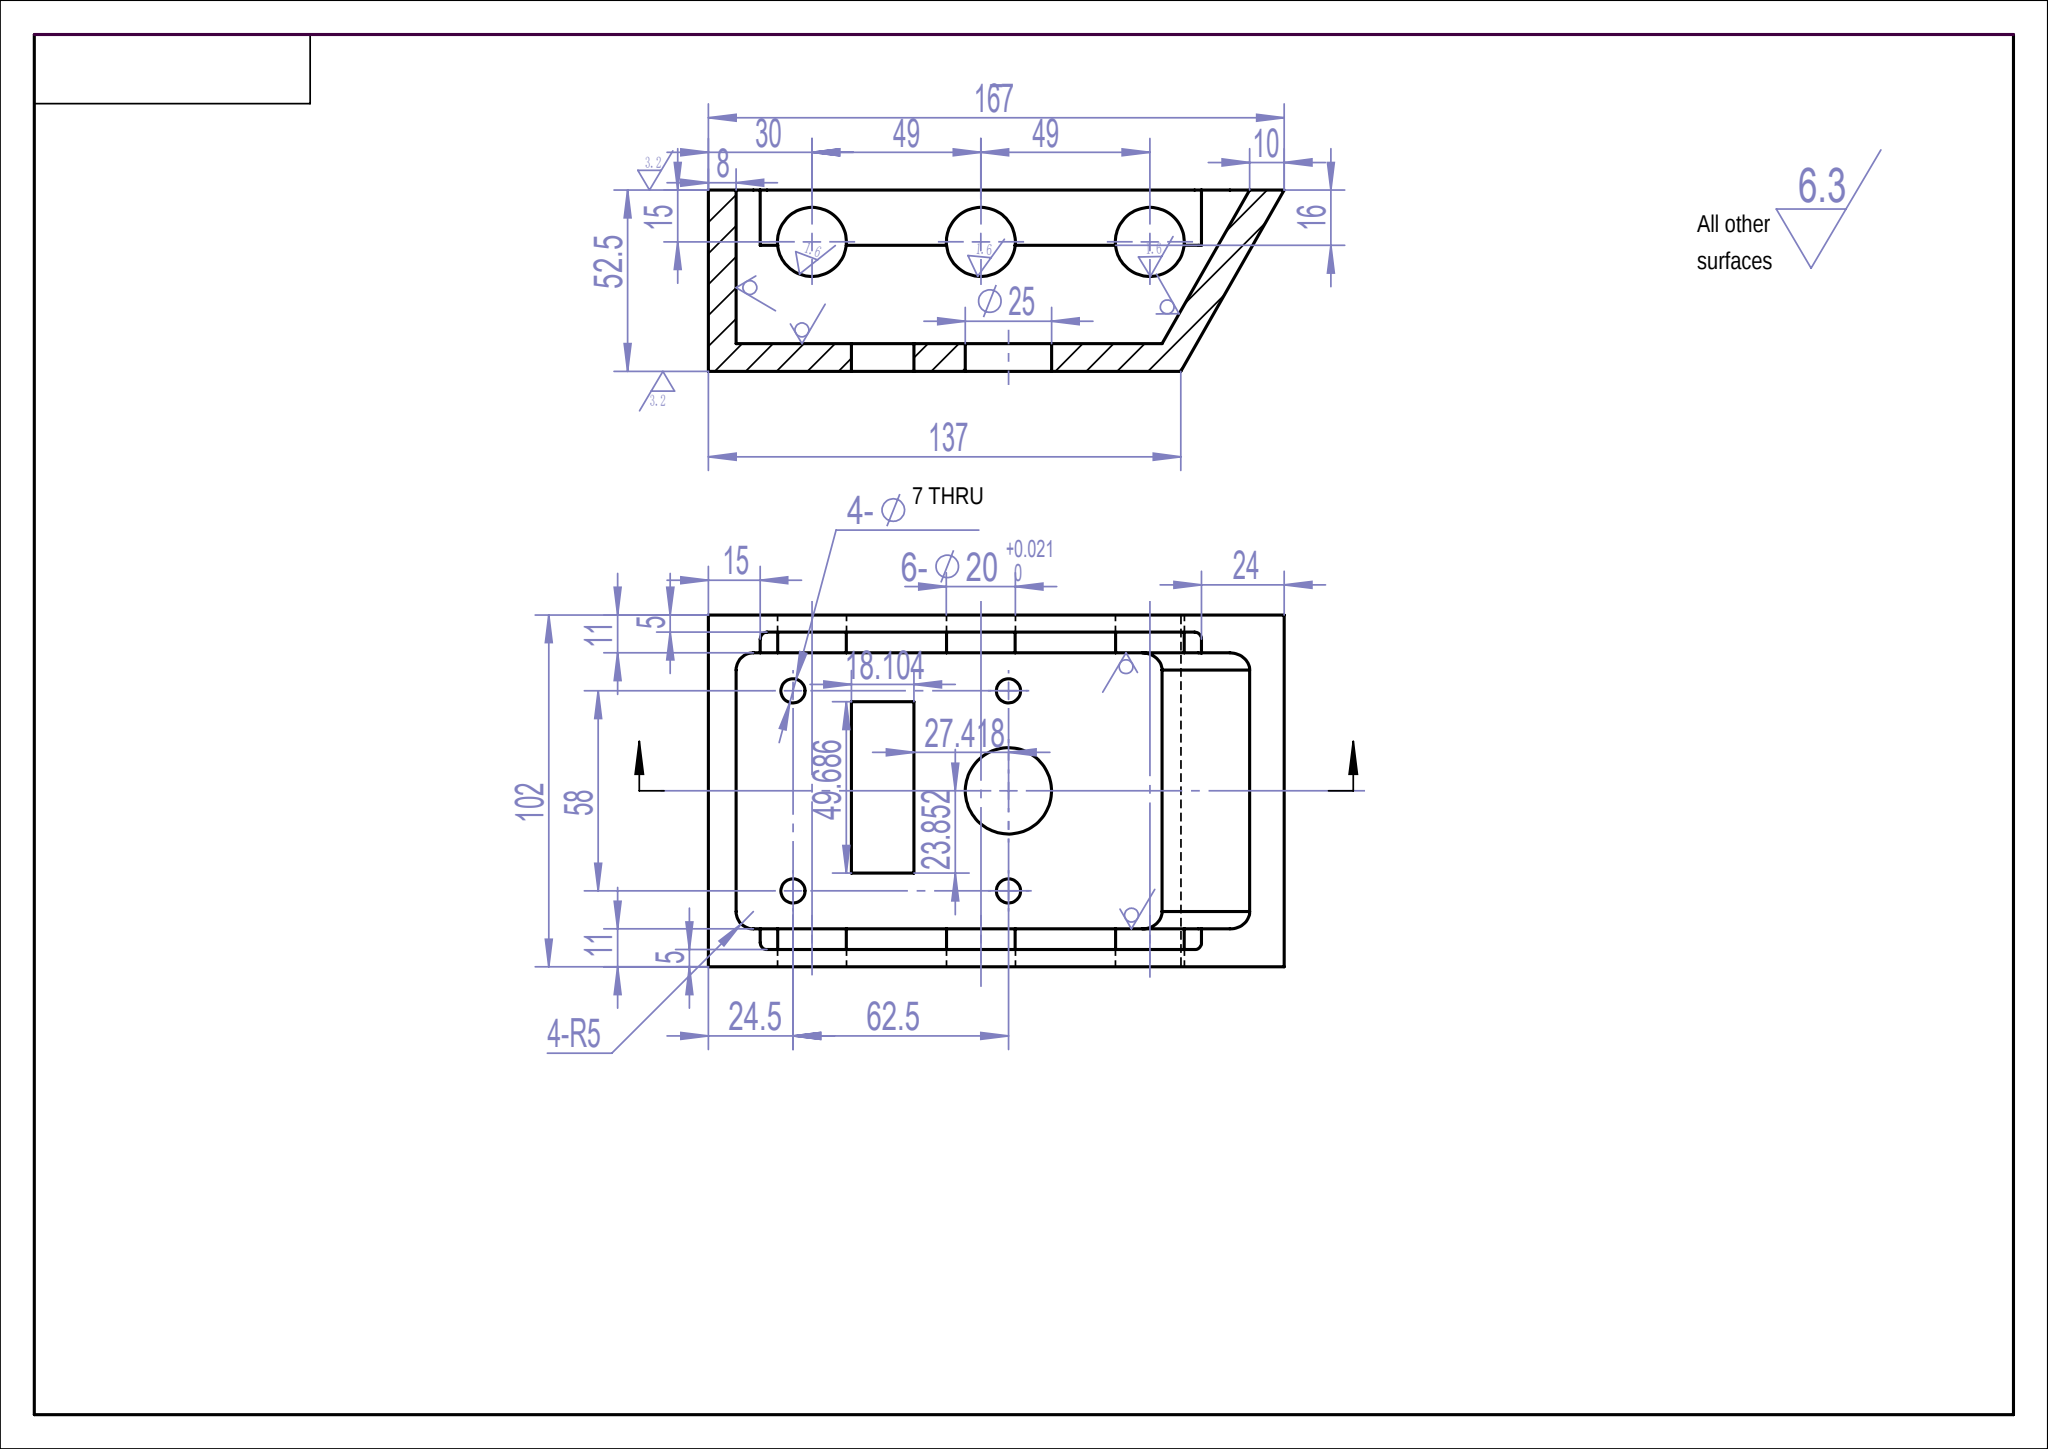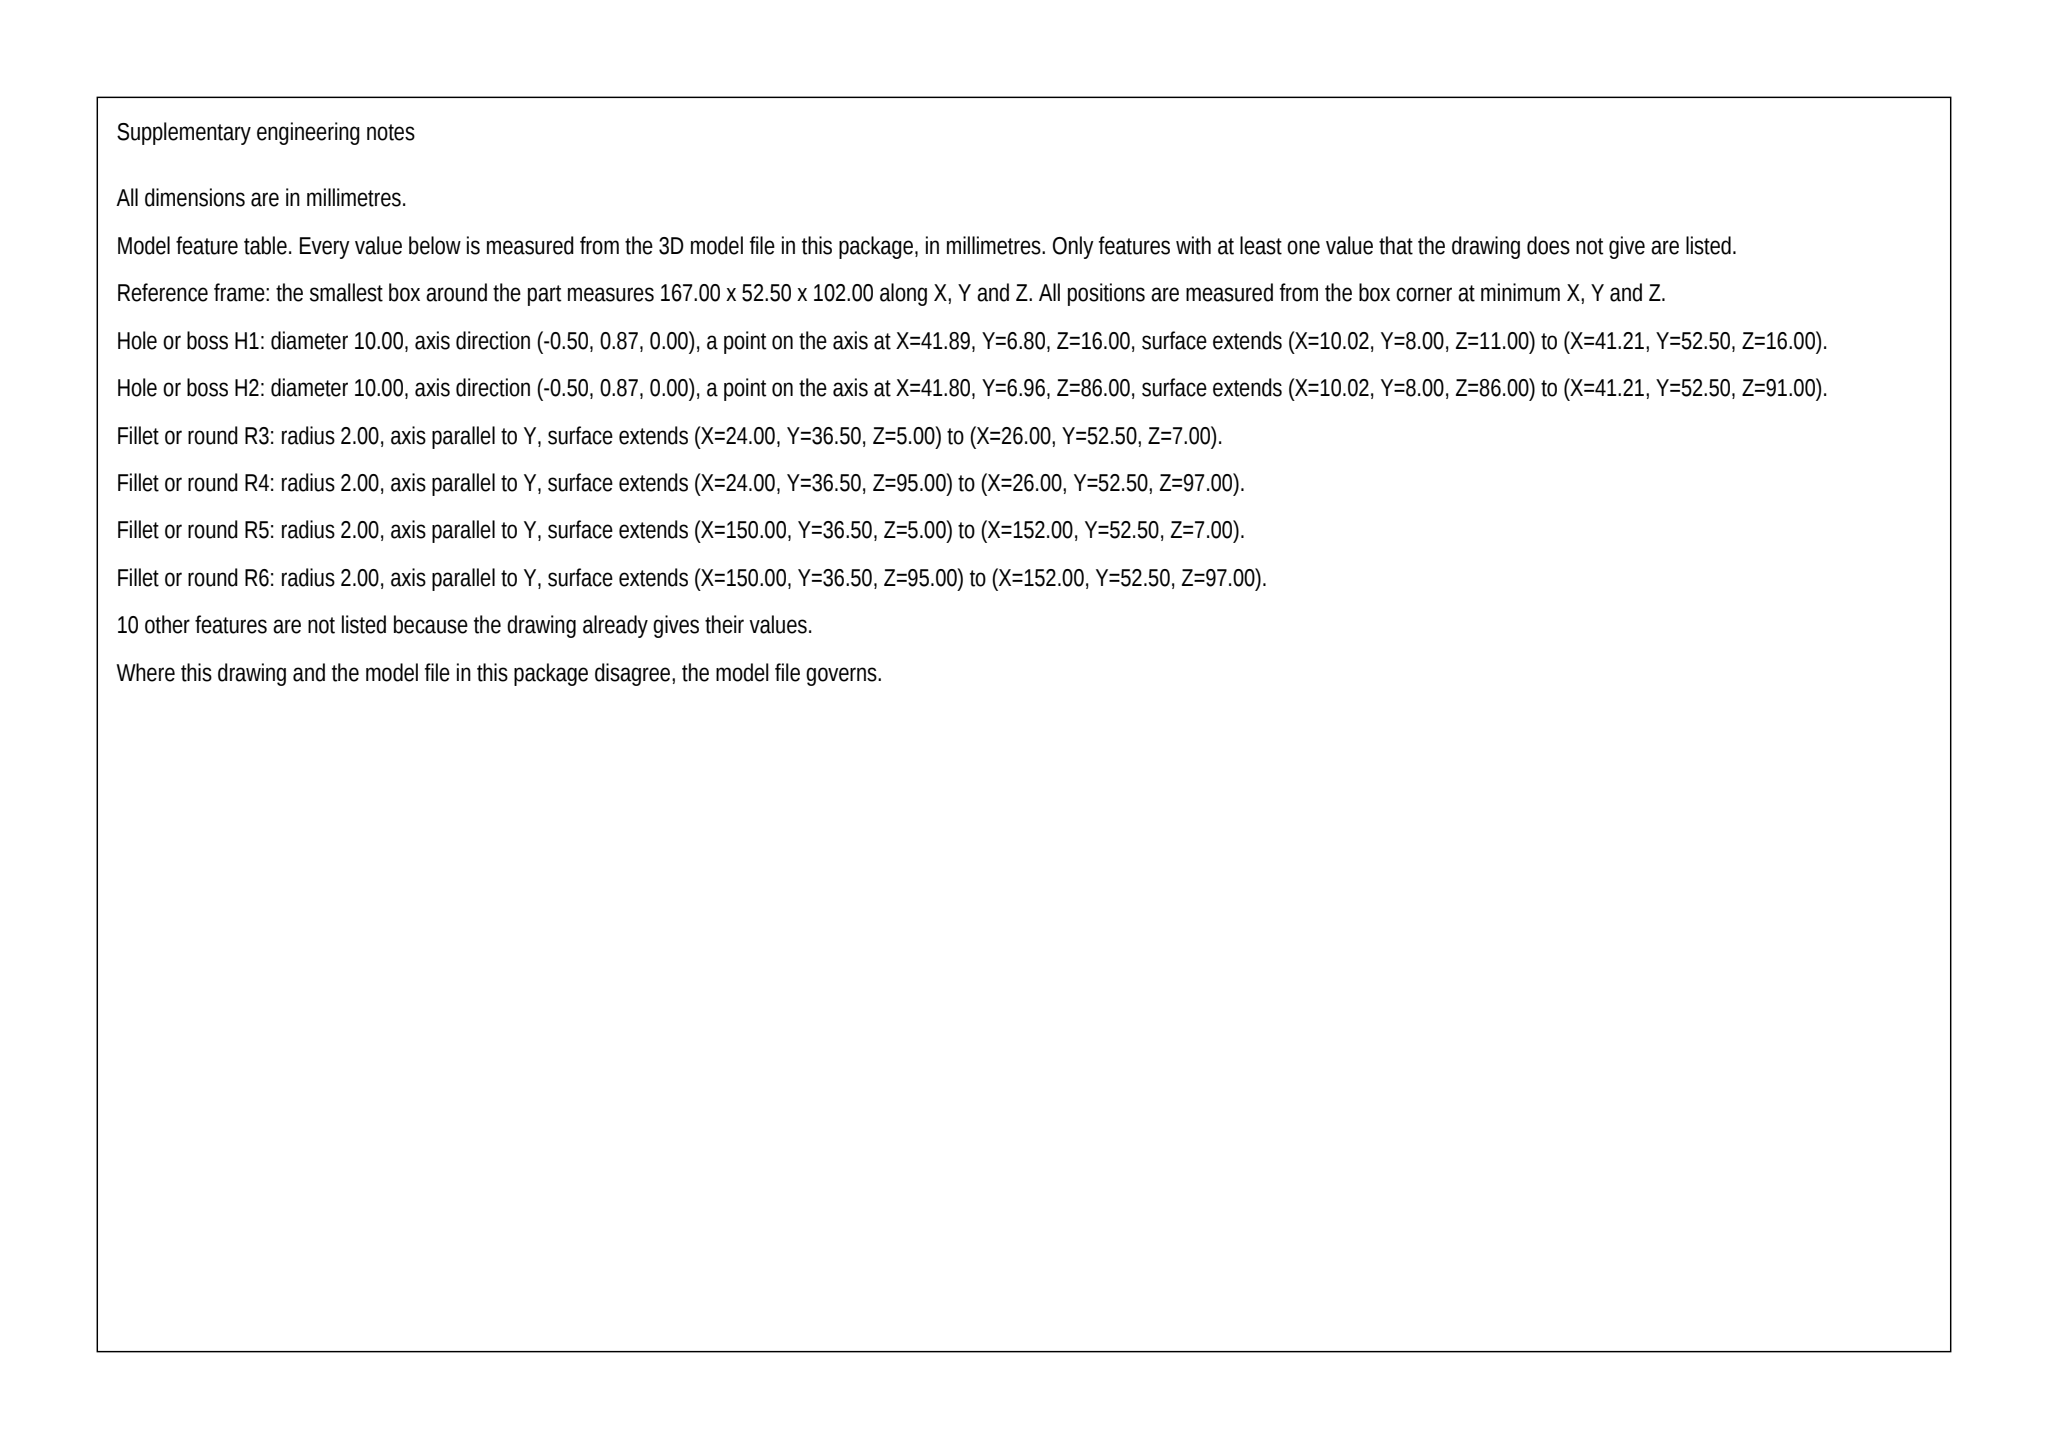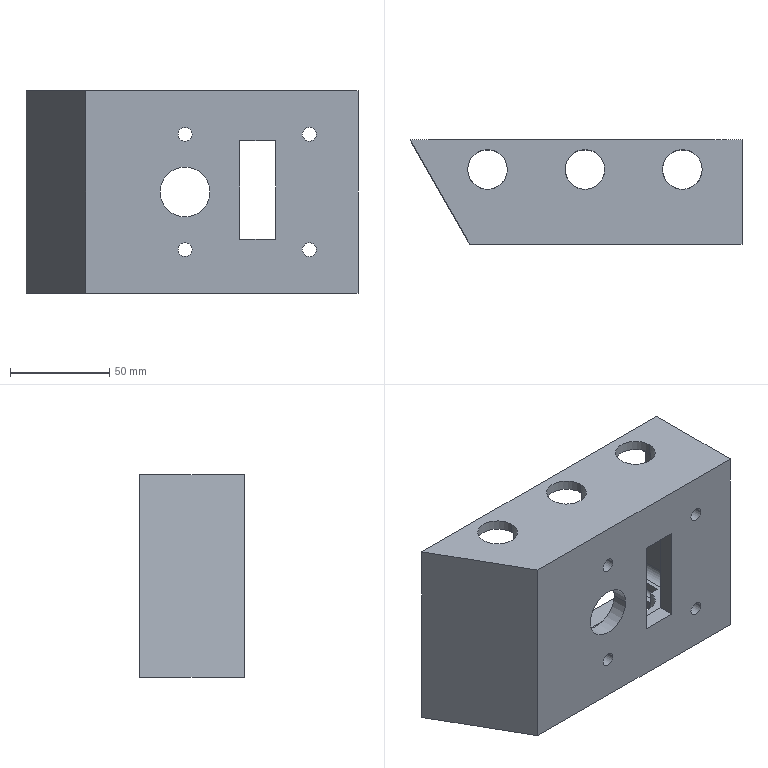Part | SolidWorks | mm | 1 solid | 61 faces | box 167 x 52.5 x 102 mm | volume 278646 mm3 | plane 31 | cylinder 30 | commonest cylinder face diameters 20 x12 7 x8 10 x4 4 x4 25 x2